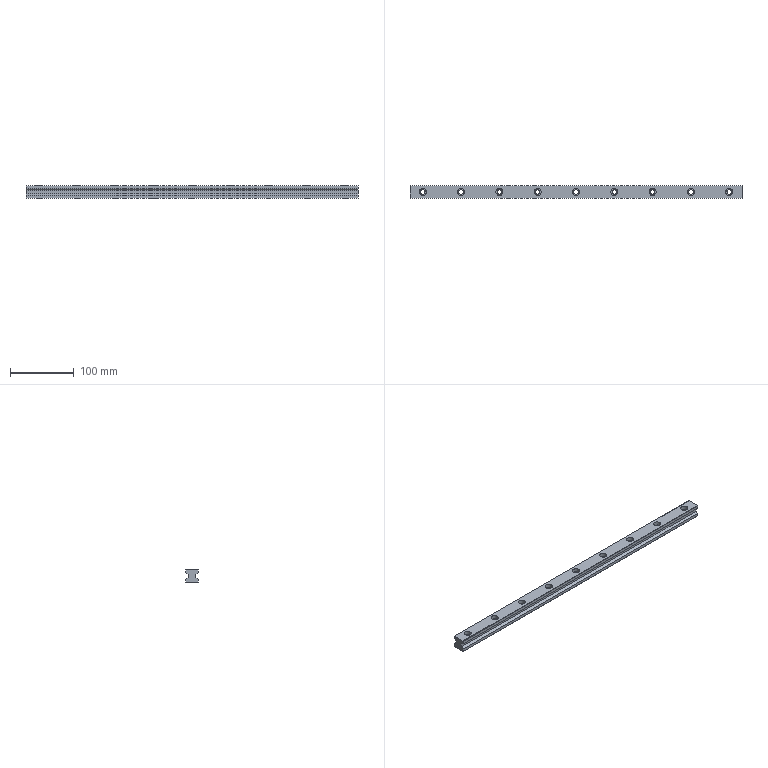Component | NX | LINEAR_GUIDE_RAIL_2 | 1 solid | 45 faces | volume 165766 mm3 | plane 27 | cylinder 18 | commonest cylinder face diameters 7 x9 11 x9